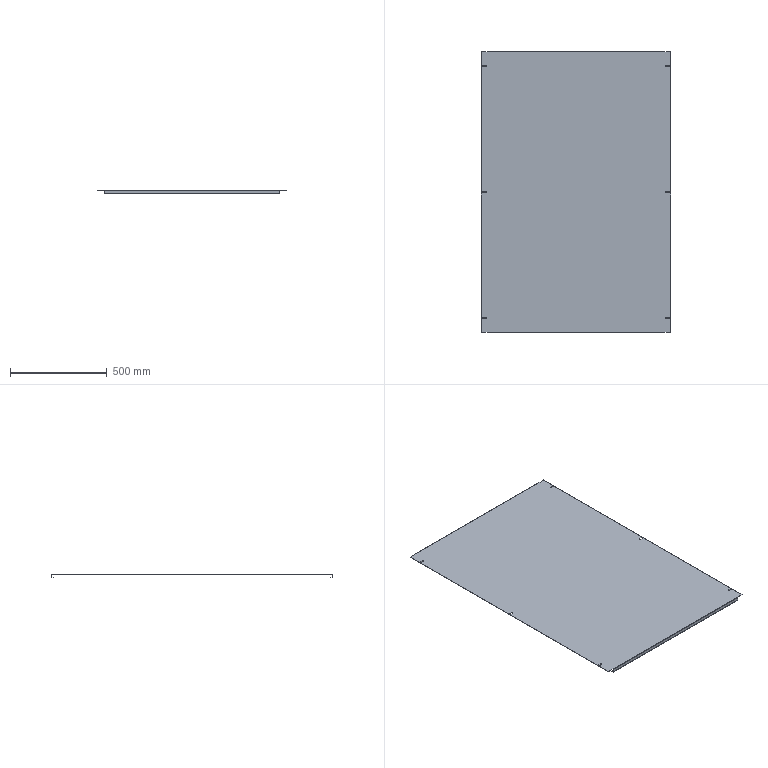Component | SolidWorks | AirFurnaceElectricalCabinet-ElectricalPanelAssembly-1_AirFurnaceElectricalCabinet-ElectricalPanel-1 | 1 solid | 72 faces | volume 2194075 mm3 | plane 46 | cylinder 26 | commonest cylinder face diameters 8 x18 1.5 x4 4.5 x4